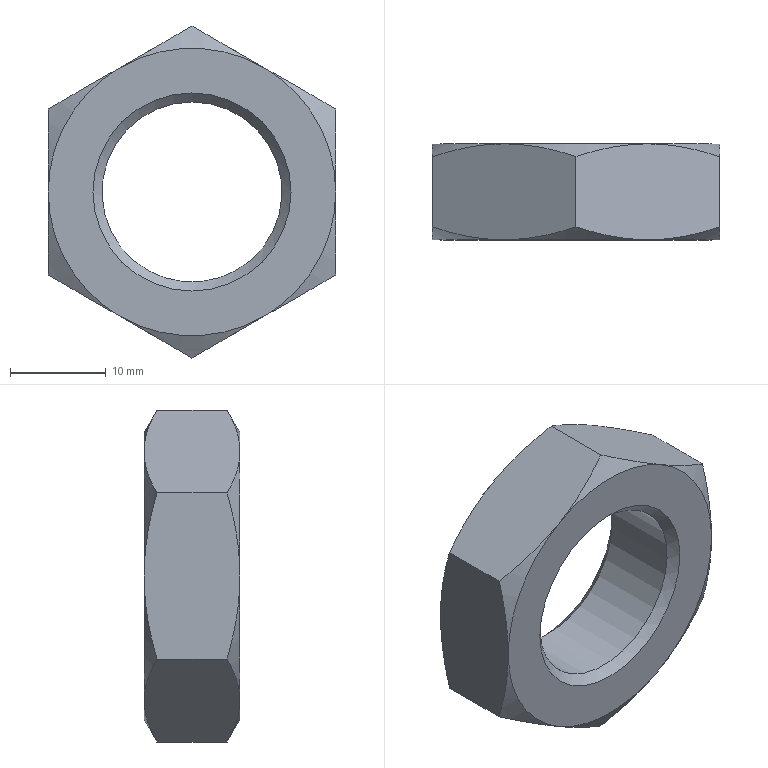Component | NX | GB-T6173-2000_M20X1_5 | 1 solid | 23 faces | volume 4910 mm3 | cone 14 | plane 8 | cylinder 1 | commonest cylinder face diameters 18.782 x1